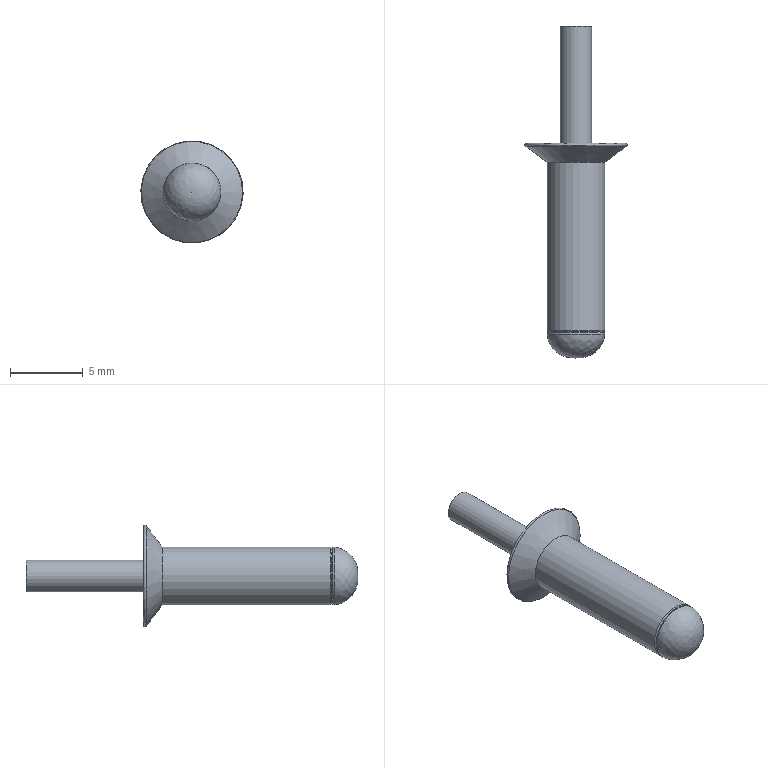Component | NX | DOWEL_PIN | 1 solid | 12 faces | box 7.06 x 22.89 x 7.06 mm | volume 221 mm3 | plane 3 | cylinder 3 | torus 3 | cone 2 | spline 1 | commonest cylinder face diameters 2.174 x1 3.478 x1 4 x1
STEP:
#1=CARTESIAN_POINT('',(0.,0.,0.));
#2=DIRECTION('',(0.,0.,1.));
#3=DIRECTION('',(1.,0.,0.));
#4=AXIS2_PLACEMENT_3D('',#1,#2,#3);
#5=CARTESIAN_POINT('',(-163.683,14.404,282.582));
#6=VERTEX_POINT('',#5);
#7=CARTESIAN_POINT('',(-164.277,14.404,283.491));
#8=DIRECTION('',(0.,1.,0.));
#9=DIRECTION('',(0.5469,0.,-0.8372));
#10=AXIS2_PLACEMENT_3D('',#7,#8,#9);
#11=CIRCLE('',#10,1.087);
#12=CARTESIAN_POINT('',(-164.277,14.404,283.491));
#13=DIRECTION('',(0.,1.,0.));
#14=DIRECTION('',(0.5469,0.,-0.8372));
#15=AXIS2_PLACEMENT_3D('',#12,#13,#14);
#16=PLANE('',#15);
#17=CARTESIAN_POINT('',(-0.,0.));
#18=DIRECTION('',(1.,-0.));
#19=AXIS2_PLACEMENT_2D('',#17,#18);
#20=CIRCLE('',#19,1.087);
#21=(GEOMETRIC_REPRESENTATION_CONTEXT(2)PARAMETRIC_REPRESENTATION_CONTEXT()REPRESENTATION_CONTEXT('',''));
#22=DEFINITIONAL_REPRESENTATION('',(#20),#21);
#23=PCURVE('',#16,#22);
#24=CARTESIAN_POINT('',(-164.277,36.087,283.491));
#25=DIRECTION('',(0.,1.,0.));
#26=DIRECTION('',(0.5469,0.,-0.8372));
#27=AXIS2_PLACEMENT_3D('',#24,#25,#26);
#28=CYLINDRICAL_SURFACE('',#27,1.087);
#29=CARTESIAN_POINT('',(0.,-21.684));
#30=DIRECTION('',(1.,0.));
#31=VECTOR('',#30,1.);
#32=LINE('',#29,#31);
#33=(GEOMETRIC_REPRESENTATION_CONTEXT(2)PARAMETRIC_REPRESENTATION_CONTEXT()REPRESENTATION_CONTEXT('',''));
#34=DEFINITIONAL_REPRESENTATION('',(#32),#33);
#35=PCURVE('',#28,#34);
#36=SURFACE_CURVE('',#11,(#23,#35),.PCURVE_S1.);
#37=EDGE_CURVE('',#6,#6,#36,.T.);
#38=ORIENTED_EDGE('',*,*,#37,.T.);
#39=EDGE_LOOP('',(#38));
#40=FACE_BOUND('',#39,.T.);
#41=ADVANCED_FACE('',(#40),#16,.T.);
#42=CARTESIAN_POINT('',(-163.683,5.348,282.582));
#43=VERTEX_POINT('',#42);
#44=CARTESIAN_POINT('',(-164.277,5.348,283.491));
#45=DIRECTION('',(0.,1.,0.));
#46=DIRECTION('',(0.5469,0.,-0.8372));
#47=AXIS2_PLACEMENT_3D('',#44,#45,#46);
#48=CIRCLE('',#47,1.087);
#49=CARTESIAN_POINT('',(0.,-30.74));
#50=DIRECTION('',(1.,0.));
#51=VECTOR('',#50,1.);
#52=LINE('',#49,#51);
#53=(GEOMETRIC_REPRESENTATION_CONTEXT(2)PARAMETRIC_REPRESENTATION_CONTEXT()REPRESENTATION_CONTEXT('',''));
#54=DEFINITIONAL_REPRESENTATION('',(#52),#53);
#55=PCURVE('',#28,#54);
#56=CARTESIAN_POINT('',(-165.187,5.348,282.897));
#57=DIRECTION('',(0.,1.,0.));
#58=DIRECTION('',(0.5469,0.,-0.8372));
#59=AXIS2_PLACEMENT_3D('',#56,#57,#58);
#60=PLANE('',#59);
#61=CARTESIAN_POINT('',(-0.,-1.087));
#62=DIRECTION('',(1.,-0.));
#63=AXIS2_PLACEMENT_2D('',#61,#62);
#64=CIRCLE('',#63,1.087);
#65=(GEOMETRIC_REPRESENTATION_CONTEXT(2)PARAMETRIC_REPRESENTATION_CONTEXT()REPRESENTATION_CONTEXT('',''));
#66=DEFINITIONAL_REPRESENTATION('',(#64),#65);
#67=PCURVE('',#60,#66);
#68=SURFACE_CURVE('',#48,(#55,#67),.PCURVE_S1.);
#69=EDGE_CURVE('',#43,#43,#68,.T.);
#70=ORIENTED_EDGE('',*,*,#69,.T.);
#71=CARTESIAN_POINT('',(-163.683,5.348,282.582));
#72=CARTESIAN_POINT('',(-163.683,14.404,282.582));
#73=B_SPLINE_CURVE_WITH_KNOTS('',1,(#71,#72),.UNSPECIFIED.,.F.,.F.,(2,2),(-30.74,-21.684),.PIECEWISE_BEZIER_KNOTS.);
#74=CARTESIAN_POINT('',(6.283,0.));
#75=DIRECTION('',(0.,1.));
#76=VECTOR('',#75,1.);
#77=LINE('',#74,#76);
#78=(GEOMETRIC_REPRESENTATION_CONTEXT(2)PARAMETRIC_REPRESENTATION_CONTEXT()REPRESENTATION_CONTEXT('',''));
#79=DEFINITIONAL_REPRESENTATION('',(#77),#78);
#80=PCURVE('',#28,#79);
#81=CARTESIAN_POINT('',(0.,0.));
#82=DIRECTION('',(0.,1.));
#83=VECTOR('',#82,1.);
#84=LINE('',#81,#83);
#85=(GEOMETRIC_REPRESENTATION_CONTEXT(2)PARAMETRIC_REPRESENTATION_CONTEXT()REPRESENTATION_CONTEXT('',''));
#86=DEFINITIONAL_REPRESENTATION('',(#84),#85);
#87=PCURVE('',#28,#86);
#88=SEAM_CURVE('',#73,(#80,#87),.PCURVE_S1.);
#89=EDGE_CURVE('',#43,#6,#88,.T.);
#90=ORIENTED_EDGE('',*,*,#89,.T.);
#91=ORIENTED_EDGE('',*,*,#37,.F.);
#92=ORIENTED_EDGE('',*,*,#89,.F.);
#93=EDGE_LOOP('',(#70,#90,#91,#92));
#94=FACE_BOUND('',#93,.T.);
#95=ADVANCED_FACE('',(#94),#28,.T.);
#96=CARTESIAN_POINT('',(-163.326,5.348,282.036));
#97=VERTEX_POINT('',#96);
#98=CARTESIAN_POINT('',(-164.277,5.348,283.491));
#99=DIRECTION('',(0.,1.,0.));
#100=DIRECTION('',(0.5469,0.,-0.8372));
#101=AXIS2_PLACEMENT_3D('',#98,#99,#100);
#102=CIRCLE('',#101,1.739);
#103=CARTESIAN_POINT('',(-0.,-1.087));
#104=DIRECTION('',(1.,0.));
#105=AXIS2_PLACEMENT_2D('',#103,#104);
#106=CIRCLE('',#105,1.739);
#107=(GEOMETRIC_REPRESENTATION_CONTEXT(2)PARAMETRIC_REPRESENTATION_CONTEXT()REPRESENTATION_CONTEXT('',''));
#108=DEFINITIONAL_REPRESENTATION('',(#106),#107);
#109=PCURVE('',#60,#108);
#110=CARTESIAN_POINT('',(-164.277,36.087,283.491));
#111=DIRECTION('',(0.,1.,0.));
#112=DIRECTION('',(0.5469,0.,-0.8372));
#113=AXIS2_PLACEMENT_3D('',#110,#111,#112);
#114=CYLINDRICAL_SURFACE('',#113,1.739);
#115=CARTESIAN_POINT('',(0.,-30.74));
#116=DIRECTION('',(1.,0.));
#117=VECTOR('',#116,1.);
#118=LINE('',#115,#117);
#119=(GEOMETRIC_REPRESENTATION_CONTEXT(2)PARAMETRIC_REPRESENTATION_CONTEXT()REPRESENTATION_CONTEXT('',''));
#120=DEFINITIONAL_REPRESENTATION('',(#118),#119);
#121=PCURVE('',#114,#120);
#122=SURFACE_CURVE('',#102,(#109,#121),.PCURVE_S1.);
#123=EDGE_CURVE('',#97,#97,#122,.T.);
#124=ORIENTED_EDGE('',*,*,#123,.T.);
#125=EDGE_LOOP('',(#124));
#126=FACE_BOUND('',#125,.T.);
#127=ORIENTED_EDGE('',*,*,#69,.F.);
#128=EDGE_LOOP('',(#127));
#129=FACE_BOUND('',#128,.T.);
#130=ADVANCED_FACE('',(#126,#129),#60,.T.);
#131=CARTESIAN_POINT('',(-163.326,6.304,282.036));
#132=VERTEX_POINT('',#131);
#133=CARTESIAN_POINT('',(-164.277,6.304,283.491));
#134=DIRECTION('',(0.,1.,0.));
#135=DIRECTION('',(0.5469,0.,-0.8372));
#136=AXIS2_PLACEMENT_3D('',#133,#134,#135);
#137=CIRCLE('',#136,1.739);
#138=CARTESIAN_POINT('',(0.,-29.783));
#139=DIRECTION('',(1.,0.));
#140=VECTOR('',#139,1.);
#141=LINE('',#138,#140);
#142=(GEOMETRIC_REPRESENTATION_CONTEXT(2)PARAMETRIC_REPRESENTATION_CONTEXT()REPRESENTATION_CONTEXT('',''));
#143=DEFINITIONAL_REPRESENTATION('',(#141),#142);
#144=PCURVE('',#114,#143);
#145=CARTESIAN_POINT('',(-165.733,6.304,282.54));
#146=DIRECTION('',(0.,1.,0.));
#147=DIRECTION('',(0.5469,0.,-0.8372));
#148=AXIS2_PLACEMENT_3D('',#145,#146,#147);
#149=PLANE('',#148);
#150=CARTESIAN_POINT('',(-0.,-1.739));
#151=DIRECTION('',(1.,-0.));
#152=AXIS2_PLACEMENT_2D('',#150,#151);
#153=CIRCLE('',#152,1.739);
#154=(GEOMETRIC_REPRESENTATION_CONTEXT(2)PARAMETRIC_REPRESENTATION_CONTEXT()REPRESENTATION_CONTEXT('',''));
#155=DEFINITIONAL_REPRESENTATION('',(#153),#154);
#156=PCURVE('',#149,#155);
#157=SURFACE_CURVE('',#137,(#144,#156),.PCURVE_S1.);
#158=EDGE_CURVE('',#132,#132,#157,.T.);
#159=ORIENTED_EDGE('',*,*,#158,.F.);
#160=CARTESIAN_POINT('',(-163.326,5.348,282.036));
#161=CARTESIAN_POINT('',(-163.326,6.304,282.036));
#162=B_SPLINE_CURVE_WITH_KNOTS('',1,(#160,#161),.UNSPECIFIED.,.F.,.F.,(2,2),(-30.74,-29.783),.PIECEWISE_BEZIER_KNOTS.);
#163=CARTESIAN_POINT('',(0.,0.));
#164=DIRECTION('',(0.,1.));
#165=VECTOR('',#164,1.);
#166=LINE('',#163,#165);
#167=(GEOMETRIC_REPRESENTATION_CONTEXT(2)PARAMETRIC_REPRESENTATION_CONTEXT()REPRESENTATION_CONTEXT('',''));
#168=DEFINITIONAL_REPRESENTATION('',(#166),#167);
#169=PCURVE('',#114,#168);
#170=CARTESIAN_POINT('',(6.283,0.));
#171=DIRECTION('',(0.,1.));
#172=VECTOR('',#171,1.);
#173=LINE('',#170,#172);
#174=(GEOMETRIC_REPRESENTATION_CONTEXT(2)PARAMETRIC_REPRESENTATION_CONTEXT()REPRESENTATION_CONTEXT('',''));
#175=DEFINITIONAL_REPRESENTATION('',(#173),#174);
#176=PCURVE('',#114,#175);
#177=SEAM_CURVE('',#162,(#169,#176),.PCURVE_S1.);
#178=EDGE_CURVE('',#97,#132,#177,.T.);
#179=ORIENTED_EDGE('',*,*,#178,.F.);
#180=ORIENTED_EDGE('',*,*,#123,.T.);
#181=ORIENTED_EDGE('',*,*,#178,.T.);
#182=EDGE_LOOP('',(#159,#179,#180,#181));
#183=FACE_BOUND('',#182,.F.);
#184=ADVANCED_FACE('',(#183),#114,.F.);
#185=CARTESIAN_POINT('',(-162.4,6.304,280.618));
#186=VERTEX_POINT('',#185);
#187=CARTESIAN_POINT('',(-164.277,6.304,283.491));
#188=DIRECTION('',(0.,1.,0.));
#189=DIRECTION('',(0.5469,0.,-0.8372));
#190=AXIS2_PLACEMENT_3D('',#187,#188,#189);
#191=CIRCLE('',#190,3.432);
#192=CARTESIAN_POINT('',(-0.,-1.739));
#193=DIRECTION('',(1.,0.));
#194=AXIS2_PLACEMENT_2D('',#192,#193);
#195=CIRCLE('',#194,3.432);
#196=(GEOMETRIC_REPRESENTATION_CONTEXT(2)PARAMETRIC_REPRESENTATION_CONTEXT()REPRESENTATION_CONTEXT('',''));
#197=DEFINITIONAL_REPRESENTATION('',(#195),#196);
#198=PCURVE('',#149,#197);
#199=CARTESIAN_POINT('',(-164.277,6.204,283.491));
#200=DIRECTION('',(0.,1.,0.));
#201=DIRECTION('',(0.5469,0.,-0.8372));
#202=AXIS2_PLACEMENT_3D('',#199,#200,#201);
#203=TOROIDAL_SURFACE('',#202,3.432,0.1);
#204=CARTESIAN_POINT('',(0.,7.854));
#205=DIRECTION('',(1.,0.));
#206=VECTOR('',#205,1.);
#207=LINE('',#204,#206);
#208=(GEOMETRIC_REPRESENTATION_CONTEXT(2)PARAMETRIC_REPRESENTATION_CONTEXT()REPRESENTATION_CONTEXT('',''));
#209=DEFINITIONAL_REPRESENTATION('',(#207),#208);
#210=PCURVE('',#203,#209);
#211=SURFACE_CURVE('',#191,(#198,#210),.PCURVE_S1.);
#212=EDGE_CURVE('',#186,#186,#211,.T.);
#213=ORIENTED_EDGE('',*,*,#212,.T.);
#214=EDGE_LOOP('',(#213));
#215=FACE_BOUND('',#214,.T.);
#216=ORIENTED_EDGE('',*,*,#158,.F.);
#217=EDGE_LOOP('',(#216));
#218=FACE_BOUND('',#217,.T.);
#219=ADVANCED_FACE('',(#215,#218),#149,.T.);
#220=CARTESIAN_POINT('',(-166.187,6.125,286.415));
#221=VERTEX_POINT('',#220);
#222=CARTESIAN_POINT('',(-162.367,6.125,280.568));
#223=VERTEX_POINT('',#222);
#224=CARTESIAN_POINT('',(-164.277,6.125,283.491));
#225=DIRECTION('',(0.,-1.,0.));
#226=DIRECTION('',(-0.5469,0.,0.8372));
#227=AXIS2_PLACEMENT_3D('',#224,#225,#226);
#228=CIRCLE('',#227,3.492);
#229=CARTESIAN_POINT('',(-164.277,6.304,283.491));
#230=DIRECTION('',(0.,1.,0.));
#231=DIRECTION('',(0.5469,0.,-0.8372));
#232=AXIS2_PLACEMENT_3D('',#229,#230,#231);
#233=CONICAL_SURFACE('',#232,3.731,0.925);
#234=CARTESIAN_POINT('',(3.142,-0.1799));
#235=DIRECTION('',(-1.,0.));
#236=VECTOR('',#235,1.);
#237=LINE('',#234,#236);
#238=(GEOMETRIC_REPRESENTATION_CONTEXT(2)PARAMETRIC_REPRESENTATION_CONTEXT()REPRESENTATION_CONTEXT('',''));
#239=DEFINITIONAL_REPRESENTATION('',(#237),#238);
#240=PCURVE('',#233,#239);
#241=CARTESIAN_POINT('',(3.142,5.358));
#242=DIRECTION('',(-1.,0.));
#243=VECTOR('',#242,1.);
#244=LINE('',#241,#243);
#245=(GEOMETRIC_REPRESENTATION_CONTEXT(2)PARAMETRIC_REPRESENTATION_CONTEXT()REPRESENTATION_CONTEXT('',''));
#246=DEFINITIONAL_REPRESENTATION('',(#244),#245);
#247=PCURVE('',#203,#246);
#248=SURFACE_CURVE('',#228,(#240,#247),.PCURVE_S1.);
#249=EDGE_CURVE('',#221,#223,#248,.T.);
#250=ORIENTED_EDGE('',*,*,#249,.T.);
#251=CARTESIAN_POINT('',(-163.183,5.,281.817));
#252=VERTEX_POINT('',#251);
#253=CARTESIAN_POINT('',(-163.183,5.,281.817));
#254=CARTESIAN_POINT('',(-162.367,6.125,280.568));
#255=B_SPLINE_CURVE_WITH_KNOTS('',1,(#253,#254),.UNSPECIFIED.,.F.,.F.,(2,2),(-2.167,-0.2989),.PIECEWISE_BEZIER_KNOTS.);
#256=CARTESIAN_POINT('',(0.,0.));
#257=DIRECTION('',(0.,1.));
#258=VECTOR('',#257,1.);
#259=LINE('',#256,#258);
#260=(GEOMETRIC_REPRESENTATION_CONTEXT(2)PARAMETRIC_REPRESENTATION_CONTEXT()REPRESENTATION_CONTEXT('',''));
#261=DEFINITIONAL_REPRESENTATION('',(#259),#260);
#262=PCURVE('',#233,#261);
#263=CARTESIAN_POINT('',(6.283,0.));
#264=DIRECTION('',(0.,1.));
#265=VECTOR('',#264,1.);
#266=LINE('',#263,#265);
#267=(GEOMETRIC_REPRESENTATION_CONTEXT(2)PARAMETRIC_REPRESENTATION_CONTEXT()REPRESENTATION_CONTEXT('',''));
#268=DEFINITIONAL_REPRESENTATION('',(#266),#267);
#269=PCURVE('',#233,#268);
#270=SEAM_CURVE('',#255,(#262,#269),.PCURVE_S1.);
#271=EDGE_CURVE('',#252,#223,#270,.T.);
#272=ORIENTED_EDGE('',*,*,#271,.F.);
#273=CARTESIAN_POINT('',(-164.277,5.,283.491));
#274=DIRECTION('',(0.,1.,0.));
#275=DIRECTION('',(0.5469,0.,-0.8372));
#276=AXIS2_PLACEMENT_3D('',#273,#274,#275);
#277=CIRCLE('',#276,2.);
#278=CARTESIAN_POINT('',(0.,-1.304));
#279=DIRECTION('',(1.,0.));
#280=VECTOR('',#279,1.);
#281=LINE('',#278,#280);
#282=(GEOMETRIC_REPRESENTATION_CONTEXT(2)PARAMETRIC_REPRESENTATION_CONTEXT()REPRESENTATION_CONTEXT('',''));
#283=DEFINITIONAL_REPRESENTATION('',(#281),#282);
#284=PCURVE('',#233,#283);
#285=CARTESIAN_POINT('',(-164.277,36.087,283.491));
#286=DIRECTION('',(0.,1.,0.));
#287=DIRECTION('',(0.5469,0.,-0.8372));
#288=AXIS2_PLACEMENT_3D('',#285,#286,#287);
#289=CYLINDRICAL_SURFACE('',#288,2.);
#290=CARTESIAN_POINT('',(0.,-31.087));
#291=DIRECTION('',(1.,0.));
#292=VECTOR('',#291,1.);
#293=LINE('',#290,#292);
#294=(GEOMETRIC_REPRESENTATION_CONTEXT(2)PARAMETRIC_REPRESENTATION_CONTEXT()REPRESENTATION_CONTEXT('',''));
#295=DEFINITIONAL_REPRESENTATION('',(#293),#294);
#296=PCURVE('',#289,#295);
#297=SURFACE_CURVE('',#277,(#284,#296),.PCURVE_S1.);
#298=EDGE_CURVE('',#252,#252,#297,.T.);
#299=ORIENTED_EDGE('',*,*,#298,.T.);
#300=ORIENTED_EDGE('',*,*,#271,.T.);
#301=CARTESIAN_POINT('',(-164.277,6.125,283.491));
#302=DIRECTION('',(0.,-1.,0.));
#303=DIRECTION('',(-0.5469,0.,0.8372));
#304=AXIS2_PLACEMENT_3D('',#301,#302,#303);
#305=CIRCLE('',#304,3.492);
#306=CARTESIAN_POINT('',(9.425,-0.1799));
#307=DIRECTION('',(-1.,0.));
#308=VECTOR('',#307,1.);
#309=LINE('',#306,#308);
#310=(GEOMETRIC_REPRESENTATION_CONTEXT(2)PARAMETRIC_REPRESENTATION_CONTEXT()REPRESENTATION_CONTEXT('',''));
#311=DEFINITIONAL_REPRESENTATION('',(#309),#310);
#312=PCURVE('',#233,#311);
#313=CARTESIAN_POINT('',(9.425,5.358));
#314=DIRECTION('',(-1.,-0.));
#315=VECTOR('',#314,1.);
#316=LINE('',#313,#315);
#317=(GEOMETRIC_REPRESENTATION_CONTEXT(2)PARAMETRIC_REPRESENTATION_CONTEXT()REPRESENTATION_CONTEXT('',''));
#318=DEFINITIONAL_REPRESENTATION('',(#316),#317);
#319=PCURVE('',#203,#318);
#320=SURFACE_CURVE('',#305,(#312,#319),.PCURVE_S1.);
#321=EDGE_CURVE('',#223,#221,#320,.T.);
#322=ORIENTED_EDGE('',*,*,#321,.T.);
#323=EDGE_LOOP('',(#250,#272,#299,#300,#322));
#324=FACE_BOUND('',#323,.T.);
#325=ADVANCED_FACE('',(#324),#233,.T.);
#326=CARTESIAN_POINT('',(-163.183,-6.61,281.817));
#327=VERTEX_POINT('',#326);
#328=CARTESIAN_POINT('',(-164.277,-6.61,283.491));
#329=DIRECTION('',(0.,1.,0.));
#330=DIRECTION('',(0.5469,0.,-0.8372));
#331=AXIS2_PLACEMENT_3D('',#328,#329,#330);
#332=CIRCLE('',#331,2.);
#333=CARTESIAN_POINT('',(0.,-42.697));
#334=DIRECTION('',(1.,0.));
#335=VECTOR('',#334,1.);
#336=LINE('',#333,#335);
#337=(GEOMETRIC_REPRESENTATION_CONTEXT(2)PARAMETRIC_REPRESENTATION_CONTEXT()REPRESENTATION_CONTEXT('',''));
#338=DEFINITIONAL_REPRESENTATION('',(#336),#337);
#339=PCURVE('',#289,#338);
#340=CARTESIAN_POINT('',(-164.277,-6.69,283.491));
#341=DIRECTION('',(0.,1.,0.));
#342=DIRECTION('',(0.5469,0.,-0.8372));
#343=AXIS2_PLACEMENT_3D('',#340,#341,#342);
#344=TOROIDAL_SURFACE('',#343,1.993,0.08041);
#345=CARTESIAN_POINT('',(0.,7.769));
#346=DIRECTION('',(1.,-0.));
#347=VECTOR('',#346,1.);
#348=LINE('',#345,#347);
#349=(GEOMETRIC_REPRESENTATION_CONTEXT(2)PARAMETRIC_REPRESENTATION_CONTEXT()REPRESENTATION_CONTEXT('',''));
#350=DEFINITIONAL_REPRESENTATION('',(#348),#349);
#351=PCURVE('',#344,#350);
#352=SURFACE_CURVE('',#332,(#339,#351),.PCURVE_S1.);
#353=EDGE_CURVE('',#327,#327,#352,.T.);
#354=ORIENTED_EDGE('',*,*,#353,.T.);
#355=CARTESIAN_POINT('',(-163.183,-6.61,281.817));
#356=CARTESIAN_POINT('',(-163.183,5.,281.817));
#357=B_SPLINE_CURVE_WITH_KNOTS('',1,(#355,#356),.UNSPECIFIED.,.F.,.F.,(2,2),(-42.697,-31.087),.PIECEWISE_BEZIER_KNOTS.);
#358=CARTESIAN_POINT('',(6.283,0.));
#359=DIRECTION('',(0.,1.));
#360=VECTOR('',#359,1.);
#361=LINE('',#358,#360);
#362=(GEOMETRIC_REPRESENTATION_CONTEXT(2)PARAMETRIC_REPRESENTATION_CONTEXT()REPRESENTATION_CONTEXT('',''));
#363=DEFINITIONAL_REPRESENTATION('',(#361),#362);
#364=PCURVE('',#289,#363);
#365=CARTESIAN_POINT('',(0.,0.));
#366=DIRECTION('',(0.,1.));
#367=VECTOR('',#366,1.);
#368=LINE('',#365,#367);
#369=(GEOMETRIC_REPRESENTATION_CONTEXT(2)PARAMETRIC_REPRESENTATION_CONTEXT()REPRESENTATION_CONTEXT('',''));
#370=DEFINITIONAL_REPRESENTATION('',(#368),#369);
#371=PCURVE('',#289,#370);
#372=SEAM_CURVE('',#357,(#364,#371),.PCURVE_S1.);
#373=EDGE_CURVE('',#327,#252,#372,.T.);
#374=ORIENTED_EDGE('',*,*,#373,.T.);
#375=ORIENTED_EDGE('',*,*,#298,.F.);
#376=ORIENTED_EDGE('',*,*,#373,.F.);
#377=EDGE_LOOP('',(#354,#374,#375,#376));
#378=FACE_BOUND('',#377,.T.);
#379=ADVANCED_FACE('',(#378),#289,.T.);
#380=CARTESIAN_POINT('',(-163.231,-6.697,281.89));
#381=VERTEX_POINT('',#380);
#382=CARTESIAN_POINT('',(-164.277,-6.697,283.491));
#383=DIRECTION('',(0.,1.,0.));
#384=DIRECTION('',(0.5469,0.,-0.8372));
#385=AXIS2_PLACEMENT_3D('',#382,#383,#384);
#386=CIRCLE('',#385,1.913);
#387=CARTESIAN_POINT('',(0.,9.51));
#388=DIRECTION('',(1.,0.));
#389=VECTOR('',#388,1.);
#390=LINE('',#387,#389);
#391=(GEOMETRIC_REPRESENTATION_CONTEXT(2)PARAMETRIC_REPRESENTATION_CONTEXT()REPRESENTATION_CONTEXT('',''));
#392=DEFINITIONAL_REPRESENTATION('',(#390),#391);
#393=PCURVE('',#344,#392);
#394=CARTESIAN_POINT('',(-164.277,-6.697,283.491));
#395=DIRECTION('',(0.,-1.,0.));
#396=DIRECTION('',(-0.5469,0.,0.8372));
#397=AXIS2_PLACEMENT_3D('',#394,#395,#396);
#398=CONICAL_SURFACE('',#397,1.913,0.7854);
#399=CARTESIAN_POINT('',(9.425,0.));
#400=DIRECTION('',(-1.,0.));
#401=VECTOR('',#400,1.);
#402=LINE('',#399,#401);
#403=(GEOMETRIC_REPRESENTATION_CONTEXT(2)PARAMETRIC_REPRESENTATION_CONTEXT()REPRESENTATION_CONTEXT('',''));
#404=DEFINITIONAL_REPRESENTATION('',(#402),#403);
#405=PCURVE('',#398,#404);
#406=SURFACE_CURVE('',#386,(#393,#405),.PCURVE_S1.);
#407=EDGE_CURVE('',#381,#381,#406,.T.);
#408=ORIENTED_EDGE('',*,*,#407,.F.);
#409=CARTESIAN_POINT('',(-163.183,-6.61,281.817));
#410=CARTESIAN_POINT('',(-163.197,-6.608,281.837));
#411=CARTESIAN_POINT('',(-163.21,-6.614,281.857));
#412=CARTESIAN_POINT('',(-163.221,-6.628,281.874));
#413=CARTESIAN_POINT('',(-163.229,-6.649,281.886));
#414=CARTESIAN_POINT('',(-163.232,-6.673,281.892));
#415=CARTESIAN_POINT('',(-163.231,-6.697,281.89));
#416=(BOUNDED_CURVE()B_SPLINE_CURVE(6,(#409,#410,#411,#412,#413,#414,#415),.UNSPECIFIED.,.F.,.F.)B_SPLINE_CURVE_WITH_KNOTS((7,7),(1.486,3.227),.PIECEWISE_BEZIER_KNOTS.)CURVE()GEOMETRIC_REPRESENTATION_ITEM()RATIONAL_B_SPLINE_CURVE((1.039,1.012,0.9975,0.9926,0.9975,1.012,1.039))REPRESENTATION_ITEM(''));
#417=CARTESIAN_POINT('',(0.,6.283));
#418=DIRECTION('',(0.,1.));
#419=VECTOR('',#418,1.);
#420=LINE('',#417,#419);
#421=(GEOMETRIC_REPRESENTATION_CONTEXT(2)PARAMETRIC_REPRESENTATION_CONTEXT()REPRESENTATION_CONTEXT('',''));
#422=DEFINITIONAL_REPRESENTATION('',(#420),#421);
#423=PCURVE('',#344,#422);
#424=CARTESIAN_POINT('',(6.283,6.283));
#425=DIRECTION('',(0.,1.));
#426=VECTOR('',#425,1.);
#427=LINE('',#424,#426);
#428=(GEOMETRIC_REPRESENTATION_CONTEXT(2)PARAMETRIC_REPRESENTATION_CONTEXT()REPRESENTATION_CONTEXT('',''));
#429=DEFINITIONAL_REPRESENTATION('',(#427),#428);
#430=PCURVE('',#344,#429);
#431=SEAM_CURVE('',#416,(#423,#430),.PCURVE_S1.);
#432=EDGE_CURVE('',#327,#381,#431,.T.);
#433=ORIENTED_EDGE('',*,*,#432,.F.);
#434=ORIENTED_EDGE('',*,*,#353,.T.);
#435=ORIENTED_EDGE('',*,*,#432,.T.);
#436=EDGE_LOOP('',(#408,#433,#434,#435));
#437=FACE_BOUND('',#436,.F.);
#438=ADVANCED_FACE('',(#437),#344,.F.);
#439=CARTESIAN_POINT('',(-163.206,-6.742,281.852));
#440=VERTEX_POINT('',#439);
#441=CARTESIAN_POINT('',(-164.277,-6.742,283.491));
#442=DIRECTION('',(0.,1.,0.));
#443=DIRECTION('',(0.5469,0.,-0.8372));
#444=AXIS2_PLACEMENT_3D('',#441,#442,#443);
#445=CIRCLE('',#444,1.959);
#446=CARTESIAN_POINT('',(9.425,0.04551));
#447=DIRECTION('',(-1.,0.));
#448=VECTOR('',#447,1.);
#449=LINE('',#446,#448);
#450=(GEOMETRIC_REPRESENTATION_CONTEXT(2)PARAMETRIC_REPRESENTATION_CONTEXT()REPRESENTATION_CONTEXT('',''));
#451=DEFINITIONAL_REPRESENTATION('',(#449),#450);
#452=PCURVE('',#398,#451);
#453=CARTESIAN_POINT('',(-164.277,-6.829,283.491));
#454=DIRECTION('',(0.,1.,0.));
#455=DIRECTION('',(0.5469,0.,-0.8372));
#456=AXIS2_PLACEMENT_3D('',#453,#454,#455);
#457=TOROIDAL_SURFACE('',#456,1.871,0.1233);
#458=CARTESIAN_POINT('',(0.,7.069));
#459=DIRECTION('',(1.,0.));
#460=VECTOR('',#459,1.);
#461=LINE('',#458,#460);
#462=(GEOMETRIC_REPRESENTATION_CONTEXT(2)PARAMETRIC_REPRESENTATION_CONTEXT()REPRESENTATION_CONTEXT('',''));
#463=DEFINITIONAL_REPRESENTATION('',(#461),#462);
#464=PCURVE('',#457,#463);
#465=SURFACE_CURVE('',#445,(#452,#464),.PCURVE_S1.);
#466=EDGE_CURVE('',#440,#440,#465,.T.);
#467=ORIENTED_EDGE('',*,*,#466,.T.);
#468=CARTESIAN_POINT('',(-163.231,-6.697,281.89));
#469=CARTESIAN_POINT('',(-163.206,-6.742,281.852));
#470=B_SPLINE_CURVE_WITH_KNOTS('',1,(#468,#469),.UNSPECIFIED.,.F.,.F.,(2,2),(0.,0.06436),.PIECEWISE_BEZIER_KNOTS.);
#471=CARTESIAN_POINT('',(3.142,0.));
#472=DIRECTION('',(0.,1.));
#473=VECTOR('',#472,1.);
#474=LINE('',#471,#473);
#475=(GEOMETRIC_REPRESENTATION_CONTEXT(2)PARAMETRIC_REPRESENTATION_CONTEXT()REPRESENTATION_CONTEXT('',''));
#476=DEFINITIONAL_REPRESENTATION('',(#474),#475);
#477=PCURVE('',#398,#476);
#478=CARTESIAN_POINT('',(9.425,0.));
#479=DIRECTION('',(0.,1.));
#480=VECTOR('',#479,1.);
#481=LINE('',#478,#480);
#482=(GEOMETRIC_REPRESENTATION_CONTEXT(2)PARAMETRIC_REPRESENTATION_CONTEXT()REPRESENTATION_CONTEXT('',''));
#483=DEFINITIONAL_REPRESENTATION('',(#481),#482);
#484=PCURVE('',#398,#483);
#485=SEAM_CURVE('',#470,(#477,#484),.PCURVE_S1.);
#486=EDGE_CURVE('',#381,#440,#485,.T.);
#487=ORIENTED_EDGE('',*,*,#486,.F.);
#488=ORIENTED_EDGE('',*,*,#407,.F.);
#489=ORIENTED_EDGE('',*,*,#486,.T.);
#490=EDGE_LOOP('',(#467,#487,#488,#489));
#491=FACE_BOUND('',#490,.T.);
#492=ADVANCED_FACE('',(#491),#398,.T.);
#493=CARTESIAN_POINT('',(-163.187,-6.84,281.822));
#494=VERTEX_POINT('',#493);
#495=CARTESIAN_POINT('',(-164.277,-6.84,283.491));
#496=DIRECTION('',(0.,1.,0.));
#497=DIRECTION('',(0.5469,0.,-0.8372));
#498=AXIS2_PLACEMENT_3D('',#495,#496,#497);
#499=CIRCLE('',#498,1.994);
#500=CARTESIAN_POINT('',(0.,6.2));
#501=DIRECTION('',(1.,0.));
#502=VECTOR('',#501,1.);
#503=LINE('',#500,#502);
#504=(GEOMETRIC_REPRESENTATION_CONTEXT(2)PARAMETRIC_REPRESENTATION_CONTEXT()REPRESENTATION_CONTEXT('',''));
#505=DEFINITIONAL_REPRESENTATION('',(#503),#504);
#506=PCURVE('',#457,#505);
#507=CARTESIAN_POINT('',(-163.187,-6.84,281.822));
#508=CARTESIAN_POINT('',(-166.526,-6.84,279.641));
#509=CARTESIAN_POINT('',(-168.707,-6.84,282.98));
#510=CARTESIAN_POINT('',(-165.368,-6.84,285.161));
#511=CARTESIAN_POINT('',(-162.029,-6.84,287.342));
#512=CARTESIAN_POINT('',(-159.848,-6.84,284.003));
#513=CARTESIAN_POINT('',(-163.187,-6.84,281.822));
#514=CARTESIAN_POINT('',(-163.236,-7.914,281.897));
#515=CARTESIAN_POINT('',(-166.424,-7.914,279.814));
#516=CARTESIAN_POINT('',(-168.507,-7.914,283.003));
#517=CARTESIAN_POINT('',(-165.319,-7.914,285.086));
#518=CARTESIAN_POINT('',(-162.13,-7.914,287.169));
#519=CARTESIAN_POINT('',(-160.047,-7.914,283.98));
#520=CARTESIAN_POINT('',(-163.236,-7.914,281.897));
#521=CARTESIAN_POINT('',(-163.691,-8.598,282.595));
#522=CARTESIAN_POINT('',(-165.485,-8.598,281.423));
#523=CARTESIAN_POINT('',(-166.657,-8.598,283.216));
#524=CARTESIAN_POINT('',(-164.863,-8.598,284.388));
#525=CARTESIAN_POINT('',(-163.07,-8.598,285.56));
#526=CARTESIAN_POINT('',(-161.898,-8.598,283.767));
#527=CARTESIAN_POINT('',(-163.691,-8.598,282.595));
#528=CARTESIAN_POINT('',(-164.277,-8.478,283.491));
#529=CARTESIAN_POINT('',(-164.277,-8.478,283.491));
#530=CARTESIAN_POINT('',(-164.277,-8.478,283.491));
#531=CARTESIAN_POINT('',(-164.277,-8.478,283.491));
#532=CARTESIAN_POINT('',(-164.277,-8.478,283.491));
#533=CARTESIAN_POINT('',(-164.277,-8.478,283.491));
#534=CARTESIAN_POINT('',(-164.277,-8.478,283.491));
#535=(BOUNDED_SURFACE()B_SPLINE_SURFACE(3,3,((#507,#508,#509,#510,#511,#512,#513),(#514,#515,#516,#517,#518,#519,#520),(#521,#522,#523,#524,#525,#526,#527),(#528,#529,#530,#531,#532,#533,#534)),.UNSPECIFIED.,.F.,.T.,.F.)B_SPLINE_SURFACE_WITH_KNOTS((4,4),(1,3,3,3,1),(0.,1.),(-0.5,0.,0.5,1.,1.5),.UNSPECIFIED.)GEOMETRIC_REPRESENTATION_ITEM()RATIONAL_B_SPLINE_SURFACE(((1.,0.3333,0.3333,1.,0.3333,0.3333,1.),(0.7981,0.266,0.266,0.7981,0.266,0.266,0.7981),(0.7981,0.266,0.266,0.7981,0.266,0.266,0.7981),(1.,0.3333,0.3333,1.,0.3333,0.3333,1.)))REPRESENTATION_ITEM('')SURFACE());
#536=CARTESIAN_POINT('',(0.,0.));
#537=CARTESIAN_POINT('',(0.,0.02352));
#538=CARTESIAN_POINT('',(0.,0.06491));
#539=CARTESIAN_POINT('',(0.,0.1146));
#540=CARTESIAN_POINT('',(0.,0.1575));
#541=CARTESIAN_POINT('',(0.,0.196));
#542=CARTESIAN_POINT('',(0.,0.2322));
#543=CARTESIAN_POINT('',(0.,0.2678));
#544=CARTESIAN_POINT('',(0.,0.304));
#545=CARTESIAN_POINT('',(0.,0.3425));
#546=CARTESIAN_POINT('',(0.,0.3856));
#547=CARTESIAN_POINT('',(0.,0.4343));
#548=CARTESIAN_POINT('',(0.,0.5));
#549=CARTESIAN_POINT('',(0.,0.5657));
#550=CARTESIAN_POINT('',(0.,0.6144));
#551=CARTESIAN_POINT('',(0.,0.6575));
#552=CARTESIAN_POINT('',(0.,0.696));
#553=CARTESIAN_POINT('',(0.,0.7322));
#554=CARTESIAN_POINT('',(0.,0.7678));
#555=CARTESIAN_POINT('',(0.,0.804));
#556=CARTESIAN_POINT('',(0.,0.8425));
#557=CARTESIAN_POINT('',(0.,0.8854));
#558=CARTESIAN_POINT('',(0.,0.9351));
#559=CARTESIAN_POINT('',(0.,0.9765));
#560=CARTESIAN_POINT('',(0.,1.));
#561=B_SPLINE_CURVE_WITH_KNOTS('',3,(#536,#537,#538,#539,#540,#541,#542,#543,#544,#545,#546,#547,#548,#549,#550,#551,#552,#553,#554,#555,#556,#557,#558,#559,#560),.UNSPECIFIED.,.F.,.F.,(4,1,1,1,1,1,1,1,1,1,1,1,1,1,1,1,1,1,1,1,1,1,4),(0.,0.2856,0.5712,0.8568,1.142,1.428,1.714,1.999,2.285,2.57,2.856,3.142,3.427,3.713,3.998,4.284,4.57,4.855,5.141,5.426,5.712,5.998,6.283),.QUASI_UNIFORM_KNOTS.);
#562=(GEOMETRIC_REPRESENTATION_CONTEXT(2)PARAMETRIC_REPRESENTATION_CONTEXT()REPRESENTATION_CONTEXT('',''));
#563=DEFINITIONAL_REPRESENTATION('',(#561),#562);
#564=PCURVE('',#535,#563);
#565=SURFACE_CURVE('',#499,(#506,#564),.PCURVE_S1.);
#566=EDGE_CURVE('',#494,#494,#565,.T.);
#567=ORIENTED_EDGE('',*,*,#566,.T.);
#568=CARTESIAN_POINT('',(-163.187,-6.84,281.822));
#569=CARTESIAN_POINT('',(-163.185,-6.813,281.82));
#570=CARTESIAN_POINT('',(-163.188,-6.785,281.825));
#571=CARTESIAN_POINT('',(-163.196,-6.761,281.836));
#572=CARTESIAN_POINT('',(-163.206,-6.742,281.852));
#573=B_SPLINE_CURVE_WITH_KNOTS('',4,(#568,#569,#570,#571,#572),.UNSPECIFIED.,.F.,.F.,(5,5),(6.2,7.069),.PIECEWISE_BEZIER_KNOTS.);
#574=CARTESIAN_POINT('',(6.283,0.));
#575=DIRECTION('',(0.,1.));
#576=VECTOR('',#575,1.);
#577=LINE('',#574,#576);
#578=(GEOMETRIC_REPRESENTATION_CONTEXT(2)PARAMETRIC_REPRESENTATION_CONTEXT()REPRESENTATION_CONTEXT('',''));
#579=DEFINITIONAL_REPRESENTATION('',(#577),#578);
#580=PCURVE('',#457,#579);
#581=CARTESIAN_POINT('',(0.,0.));
#582=DIRECTION('',(0.,1.));
#583=VECTOR('',#582,1.);
#584=LINE('',#581,#583);
#585=(GEOMETRIC_REPRESENTATION_CONTEXT(2)PARAMETRIC_REPRESENTATION_CONTEXT()REPRESENTATION_CONTEXT('',''));
#586=DEFINITIONAL_REPRESENTATION('',(#584),#585);
#587=PCURVE('',#457,#586);
#588=SEAM_CURVE('',#573,(#580,#587),.PCURVE_S1.);
#589=EDGE_CURVE('',#494,#440,#588,.T.);
#590=ORIENTED_EDGE('',*,*,#589,.T.);
#591=ORIENTED_EDGE('',*,*,#466,.F.);
#592=ORIENTED_EDGE('',*,*,#589,.F.);
#593=EDGE_LOOP('',(#567,#590,#591,#592));
#594=FACE_BOUND('',#593,.T.);
#595=ADVANCED_FACE('',(#594),#457,.T.);
#596=CARTESIAN_POINT('',(-164.277,-8.478,283.491));
#597=VERTEX_POINT('',#596);
#598=CARTESIAN_POINT('',(-163.187,-6.84,281.822));
#599=CARTESIAN_POINT('',(-163.236,-7.914,281.897));
#600=CARTESIAN_POINT('',(-163.691,-8.598,282.595));
#601=CARTESIAN_POINT('',(-164.277,-8.478,283.491));
#602=(BOUNDED_CURVE()B_SPLINE_CURVE(3,(#598,#599,#600,#601),.UNSPECIFIED.,.F.,.F.)B_SPLINE_CURVE_WITH_KNOTS((4,4),(0.,1.),.PIECEWISE_BEZIER_KNOTS.)CURVE()GEOMETRIC_REPRESENTATION_ITEM()RATIONAL_B_SPLINE_CURVE((1.,0.7981,0.7981,1.))REPRESENTATION_ITEM(''));
#603=CARTESIAN_POINT('',(0.,1.));
#604=DIRECTION('',(1.,0.));
#605=VECTOR('',#604,1.);
#606=LINE('',#603,#605);
#607=(GEOMETRIC_REPRESENTATION_CONTEXT(2)PARAMETRIC_REPRESENTATION_CONTEXT()REPRESENTATION_CONTEXT('',''));
#608=DEFINITIONAL_REPRESENTATION('',(#606),#607);
#609=PCURVE('',#535,#608);
#610=CARTESIAN_POINT('',(0.,0.));
#611=DIRECTION('',(1.,0.));
#612=VECTOR('',#611,1.);
#613=LINE('',#610,#612);
#614=(GEOMETRIC_REPRESENTATION_CONTEXT(2)PARAMETRIC_REPRESENTATION_CONTEXT()REPRESENTATION_CONTEXT('',''));
#615=DEFINITIONAL_REPRESENTATION('',(#613),#614);
#616=PCURVE('',#535,#615);
#617=SEAM_CURVE('',#602,(#609,#616),.PCURVE_S1.);
#618=EDGE_CURVE('',#494,#597,#617,.T.);
#619=ORIENTED_EDGE('',*,*,#618,.F.);
#620=ORIENTED_EDGE('',*,*,#566,.F.);
#621=ORIENTED_EDGE('',*,*,#618,.T.);
#622=EDGE_LOOP('',(#619,#620,#621));
#623=FACE_BOUND('',#622,.T.);
#624=ADVANCED_FACE('',(#623),#535,.T.);
#625=ORIENTED_EDGE('',*,*,#249,.F.);
#626=ORIENTED_EDGE('',*,*,#321,.F.);
#627=CARTESIAN_POINT('',(-162.367,6.125,280.568));
#628=CARTESIAN_POINT('',(-162.349,6.15,280.54));
#629=CARTESIAN_POINT('',(-162.338,6.191,280.523));
#630=CARTESIAN_POINT('',(-162.339,6.242,280.525));
#631=CARTESIAN_POINT('',(-162.355,6.284,280.549));
#632=CARTESIAN_POINT('',(-162.377,6.304,280.583));
#633=CARTESIAN_POINT('',(-162.4,6.304,280.618));
#634=B_SPLINE_CURVE_WITH_KNOTS('',6,(#627,#628,#629,#630,#631,#632,#633),.UNSPECIFIED.,.F.,.F.,(7,7),(5.358,7.854),.PIECEWISE_BEZIER_KNOTS.);
#635=CARTESIAN_POINT('',(6.283,0.));
#636=DIRECTION('',(0.,1.));
#637=VECTOR('',#636,1.);
#638=LINE('',#635,#637);
#639=(GEOMETRIC_REPRESENTATION_CONTEXT(2)PARAMETRIC_REPRESENTATION_CONTEXT()REPRESENTATION_CONTEXT('',''));
#640=DEFINITIONAL_REPRESENTATION('',(#638),#639);
#641=PCURVE('',#203,#640);
#642=CARTESIAN_POINT('',(0.,0.));
#643=DIRECTION('',(0.,1.));
#644=VECTOR('',#643,1.);
#645=LINE('',#642,#644);
#646=(GEOMETRIC_REPRESENTATION_CONTEXT(2)PARAMETRIC_REPRESENTATION_CONTEXT()REPRESENTATION_CONTEXT('',''));
#647=DEFINITIONAL_REPRESENTATION('',(#645),#646);
#648=PCURVE('',#203,#647);
#649=SEAM_CURVE('',#634,(#641,#648),.PCURVE_S1.);
#650=EDGE_CURVE('',#223,#186,#649,.T.);
#651=ORIENTED_EDGE('',*,*,#650,.T.);
#652=ORIENTED_EDGE('',*,*,#212,.F.);
#653=ORIENTED_EDGE('',*,*,#650,.F.);
#654=EDGE_LOOP('',(#625,#626,#651,#652,#653));
#655=FACE_BOUND('',#654,.T.);
#656=ADVANCED_FACE('',(#655),#203,.T.);
#657=CLOSED_SHELL('',(#41,#95,#130,#184,#219,#325,#379,#438,#492,#595,#624,#656));
#658=MANIFOLD_SOLID_BREP('',#657);
#659=(LENGTH_UNIT()NAMED_UNIT(*)SI_UNIT(.MILLI.,.METRE.));
#660=UNCERTAINTY_MEASURE_WITH_UNIT(LENGTH_MEASURE(0.00001),#659,'','');
#661=(NAMED_UNIT(*)PLANE_ANGLE_UNIT()SI_UNIT($,.RADIAN.));
#662=(NAMED_UNIT(*)SI_UNIT($,.STERADIAN.)SOLID_ANGLE_UNIT());
#663=(GEOMETRIC_REPRESENTATION_CONTEXT(3)GLOBAL_UNCERTAINTY_ASSIGNED_CONTEXT((#660))GLOBAL_UNIT_ASSIGNED_CONTEXT((#659,#661,#662))REPRESENTATION_CONTEXT('',''));
#664=ADVANCED_BREP_SHAPE_REPRESENTATION('',(#4,#658),#663);